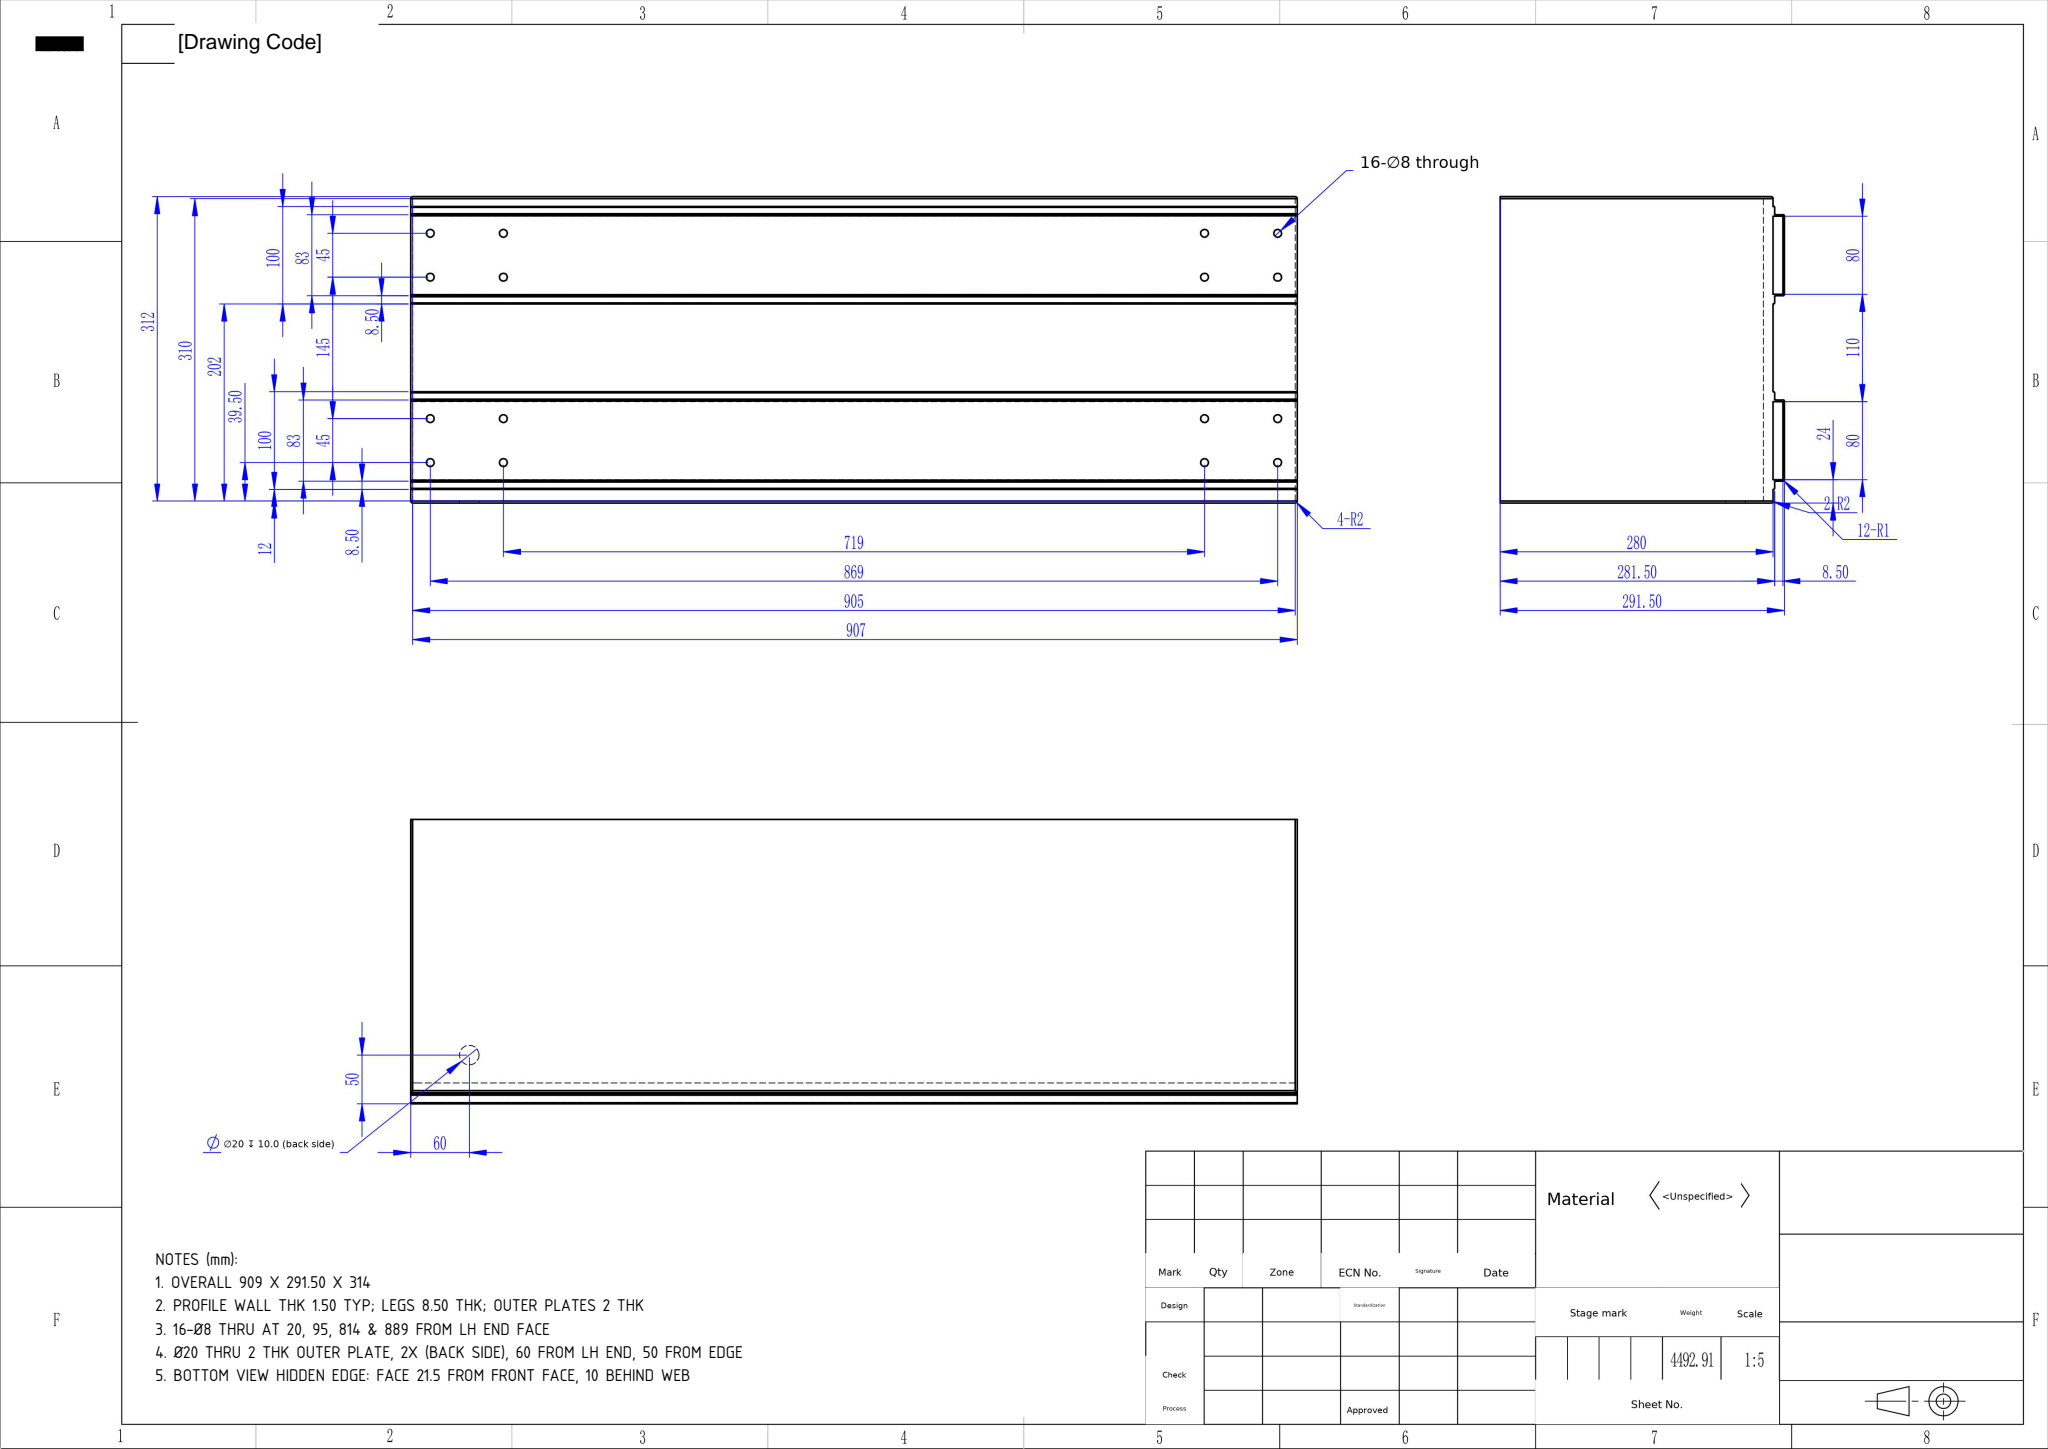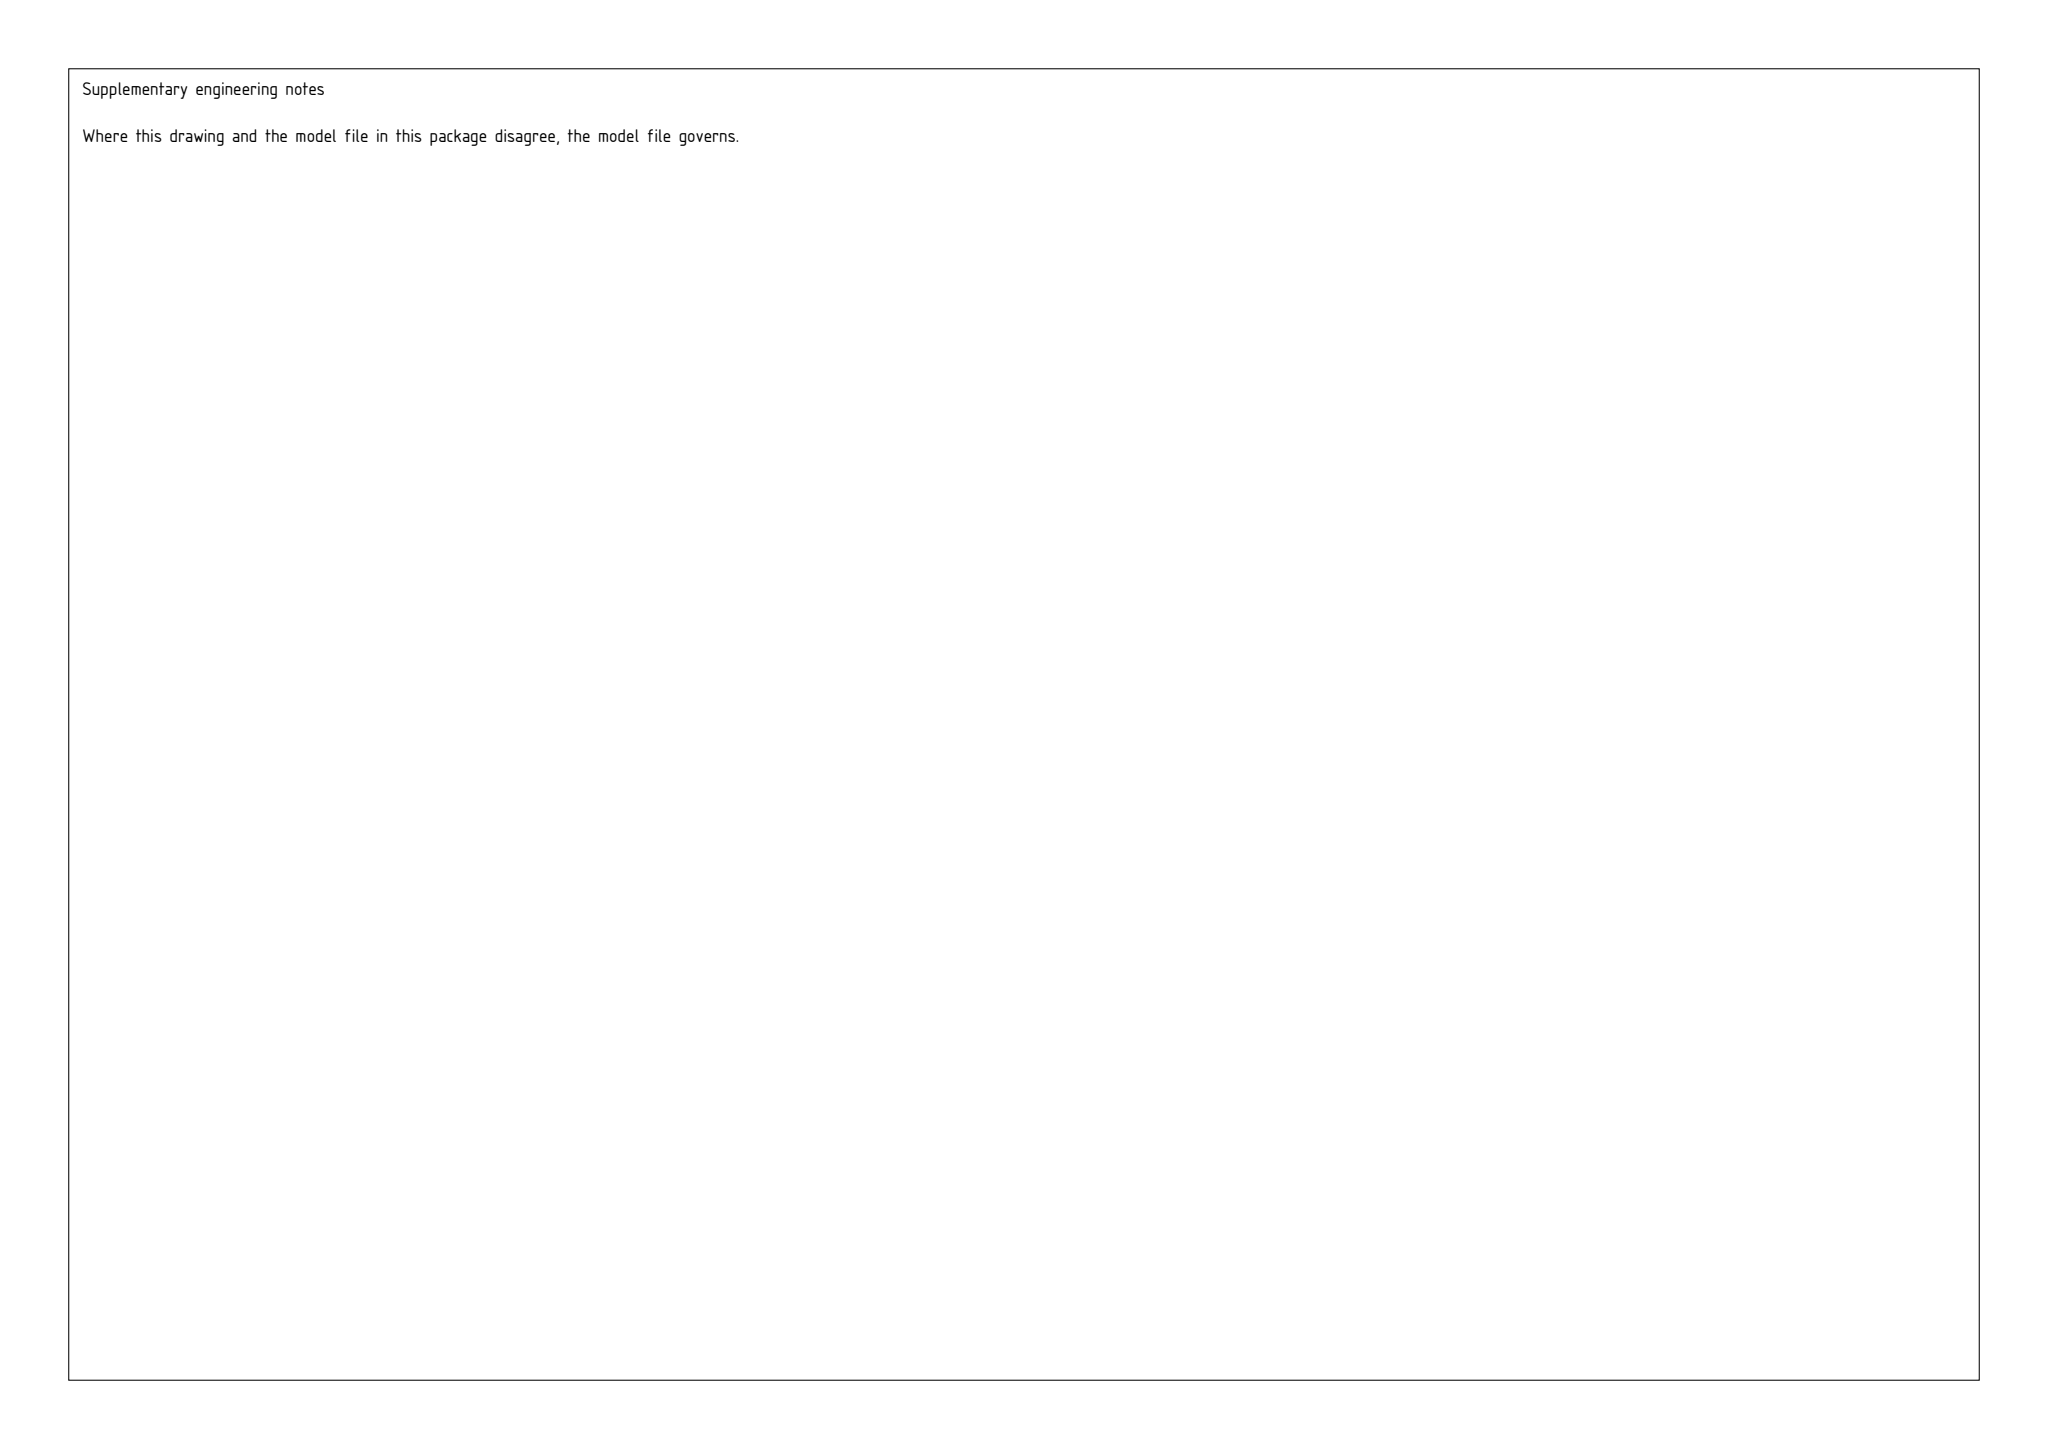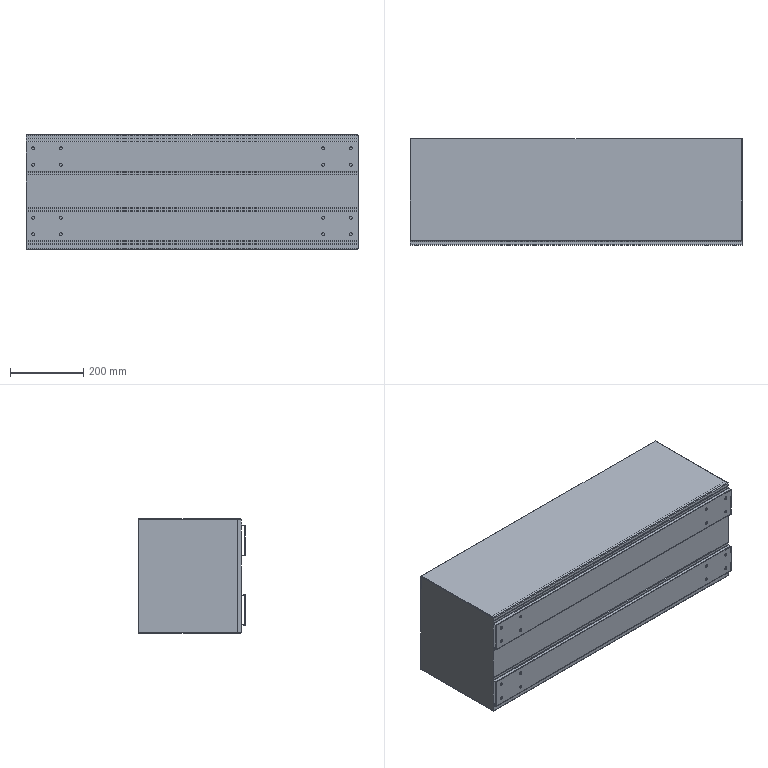Part | SolidWorks | mm | 1 solid | 87 faces | box 909 x 291.5 x 314 mm | volume 4492886 mm3 | cylinder 52 | plane 35 | commonest cylinder face diameters 8 x32 2 x12 4 x6 20 x2
Drawing notes:
OVERALL 909 X 291.50 X 314 | from the solid: bbox_xyz [909.0, 291.5, 314.0]
PROFILE WALL THK 1.50 TYP; LEGS 8.50 THK; OUTER PLATES 2 THK | from the solid: y planes 0/1.5/10/11.5 and z planes 0/2/14/22.5/24 give 1.5, 8.5 and 2 thk
16-Ø8 THRU AT 20, 95, 814 & 889 FROM LH END FACE | from the solid: Ø8 y-axis cyls at x=20, 95, 814, 889 (bbox length 909); pairs give 719 & 869
Ø20 THRU 2 THK OUTER PLATE, 2X (BACK SIDE), 60 FROM LH END, 50 FROM EDGE | from the solid: cylinders [20.0,'z',[60.0,50.0,null],2.0,count 2]; z planes 0-2 and 312-314
BOTTOM VIEW HIDDEN EDGE: FACE 21.5 FROM FRONT FACE, 10 BEHIND WEB | from the solid: axis_planes y=21.5 (1) vs web face y=11.5; 21.5-11.5=10; front face y=0
build123d program:
from build123d import *

# Parameters (mm, degrees)
SKETCH1_W               = 909
SKETCH1_H               = 314
SKETCH1_W_2             = 905
SKETCH1_H_2             = 310
BOSS_EXTRUDE1_DEPTH     = 275
SKETCH2_W               = 909
SKETCH2_H               = 314
BOSS_EXTRUDE2_DEPTH     = 5
BOSS_EXTRUDE3_DEPTH     = 909
FILLET1_R               = 1
FILLET2_R               = 1
CUT_EXTRUDE1_START      = -1.5
SKETCH5_R               = 4
CUT_EXTRUDE1_DEPTH      = 1004.98
FILLET3_R               = 2
SKETCH6_R               = 10
CUT_EXTRUDE2_DEPTH      = 10
MIRROR3_START           = -1.5
MIRROR3_COPY_1_SKETCH_R = 4
MIRROR3_COPY_1_DEPTH    = 1004.98


with BuildPart() as part:
    # Sketch1 → Boss-Extrude1 (new body)
    with BuildSketch(Plane(origin=(0, 0, 0), x_dir=(1, 0, 0), z_dir=(0, 1, 0))):
        with Locations((-452.5, 155)):
            Rectangle(SKETCH1_W, SKETCH1_H)
        with Locations((-452.5, 155)):
            Rectangle(SKETCH1_W_2, SKETCH1_H_2, mode=Mode.SUBTRACT)
    extrude(amount=BOSS_EXTRUDE1_DEPTH)

    # Sketch2 → Boss-Extrude2 (add, symmetric)
    with BuildSketch(Plane.XZ):
        with Locations((-452.5, -155)):
            Rectangle(SKETCH2_W, SKETCH2_H)
    extrude(amount=BOSS_EXTRUDE2_DEPTH, both=True)

    # Sketch4 → Boss-Extrude3 (add)
    with BuildSketch(Plane(origin=(2, 0, 0), x_dir=(0, 0, -1), z_dir=(1, 0, 0))):
        Polygon((18, -5), (8, -5), (8, -6.5), (16.5, -6.5), (16.5, -16.5), (99.5, -16.5), (99.5, -6.5), (108, -6.5), (108, -5), (98, -5), (98, -15), (18, -15), align=None)
    boss_extrude3 = extrude(amount=-BOSS_EXTRUDE3_DEPTH)

    # Fillet1
    fillet1_edges = [part.edges().sort_by_distance(p)[0] for p in [
        (-452.5, -6.5, -16.5),
        (-452.5, -6.5, -8),
        (-452.5, -6.5, -108),
        (-452.5, -6.5, -99.5),
        (-452.5, -16.5, -99.5),
        (-452.5, -16.5, -16.5),
    ]]
    fillet(fillet1_edges, radius=FILLET1_R)

    # Mirror1: Boss-Extrude3 across plane
    add(boss_extrude3.mirror(Plane.XY.offset(-153)))

    # Fillet2
    fillet2_edges = [part.edges().sort_by_distance(p)[0] for p in [
        (-452.5, -6.5, -198),
        (-452.5, -6.5, -206.5),
        (-452.5, -16.5, -206.5),
        (-452.5, -16.5, -289.5),
        (-452.5, -6.5, -289.5),
        (-452.5, -6.5, -298),
    ]]
    fillet(fillet2_edges, radius=FILLET2_R)

    # Sketch5 → Cut-Extrude1 (cut)
    with BuildSketch(Plane(origin=(0, -16.5, 0), x_dir=(-1, 0, 0), z_dir=(0, -1, 0)).offset(CUT_EXTRUDE1_START)):
        with Locations(Location((887, 270.5, 0), (0, 0, 90))):
            Circle(SKETCH5_R)
        with Locations(Location((887, 225.5, 0), (0, 0, 90))):
            Circle(SKETCH5_R)
        with Locations(Location((812, 225.5, 0), (0, 0, 90))):
            Circle(SKETCH5_R)
        with Locations(Location((812, 270.5, 0), (0, 0, 90))):
            Circle(SKETCH5_R)
    cut_extrude1 = extrude(amount=CUT_EXTRUDE1_DEPTH, mode=Mode.SUBTRACT)

    # Mirror2: Cut-Extrude1 across plane
    add(cut_extrude1.mirror(Plane.XY.offset(-153)), mode=Mode.SUBTRACT)

    # Fillet3
    fillet3_edges = [part.edges().sort_by_distance(p)[0] for p in [
        (-452.5, -5, -312),
        (-452.5, -5, 2),
        (2, 135, 2),
        (-907, 135, 2),
        (-907, 135, -312),
        (2, 135, -312),
    ]]
    fillet(fillet3_edges, radius=FILLET3_R)

    # Sketch6 → Cut-Extrude2 (cut)
    with BuildSketch(Plane(origin=(0, 0, -312), x_dir=(-1, 0, 0), z_dir=(0, 0, -1))):
        with Locations((847, 33.5)):
            Circle(SKETCH6_R)
    extrude(amount=-CUT_EXTRUDE2_DEPTH, mode=Mode.SUBTRACT)

    # Mirror3: Cut-Extrude1 across plane
    add(cut_extrude1.mirror(Plane(origin=(-452.5, 0, 0), x_dir=(0, 0, 1), z_dir=(1, 0, 0))), mode=Mode.SUBTRACT)

    # Mirror3 copy 1 sketch → Mirror3 copy 1 (cut)
    with BuildSketch(Plane(origin=(-905, -16.5, -306), x_dir=(1, 0, 0), z_dir=(0, -1, 0)).offset(MIRROR3_START)):
        with Locations(Location((887, 270.5, 0), (0, 0, 90))):
            Circle(MIRROR3_COPY_1_SKETCH_R)
        with Locations(Location((887, 225.5, 0), (0, 0, 90))):
            Circle(MIRROR3_COPY_1_SKETCH_R)
        with Locations(Location((812, 225.5, 0), (0, 0, 90))):
            Circle(MIRROR3_COPY_1_SKETCH_R)
        with Locations(Location((812, 270.5, 0), (0, 0, 90))):
            Circle(MIRROR3_COPY_1_SKETCH_R)
    extrude(amount=MIRROR3_COPY_1_DEPTH, mode=Mode.SUBTRACT)


solid = part.part